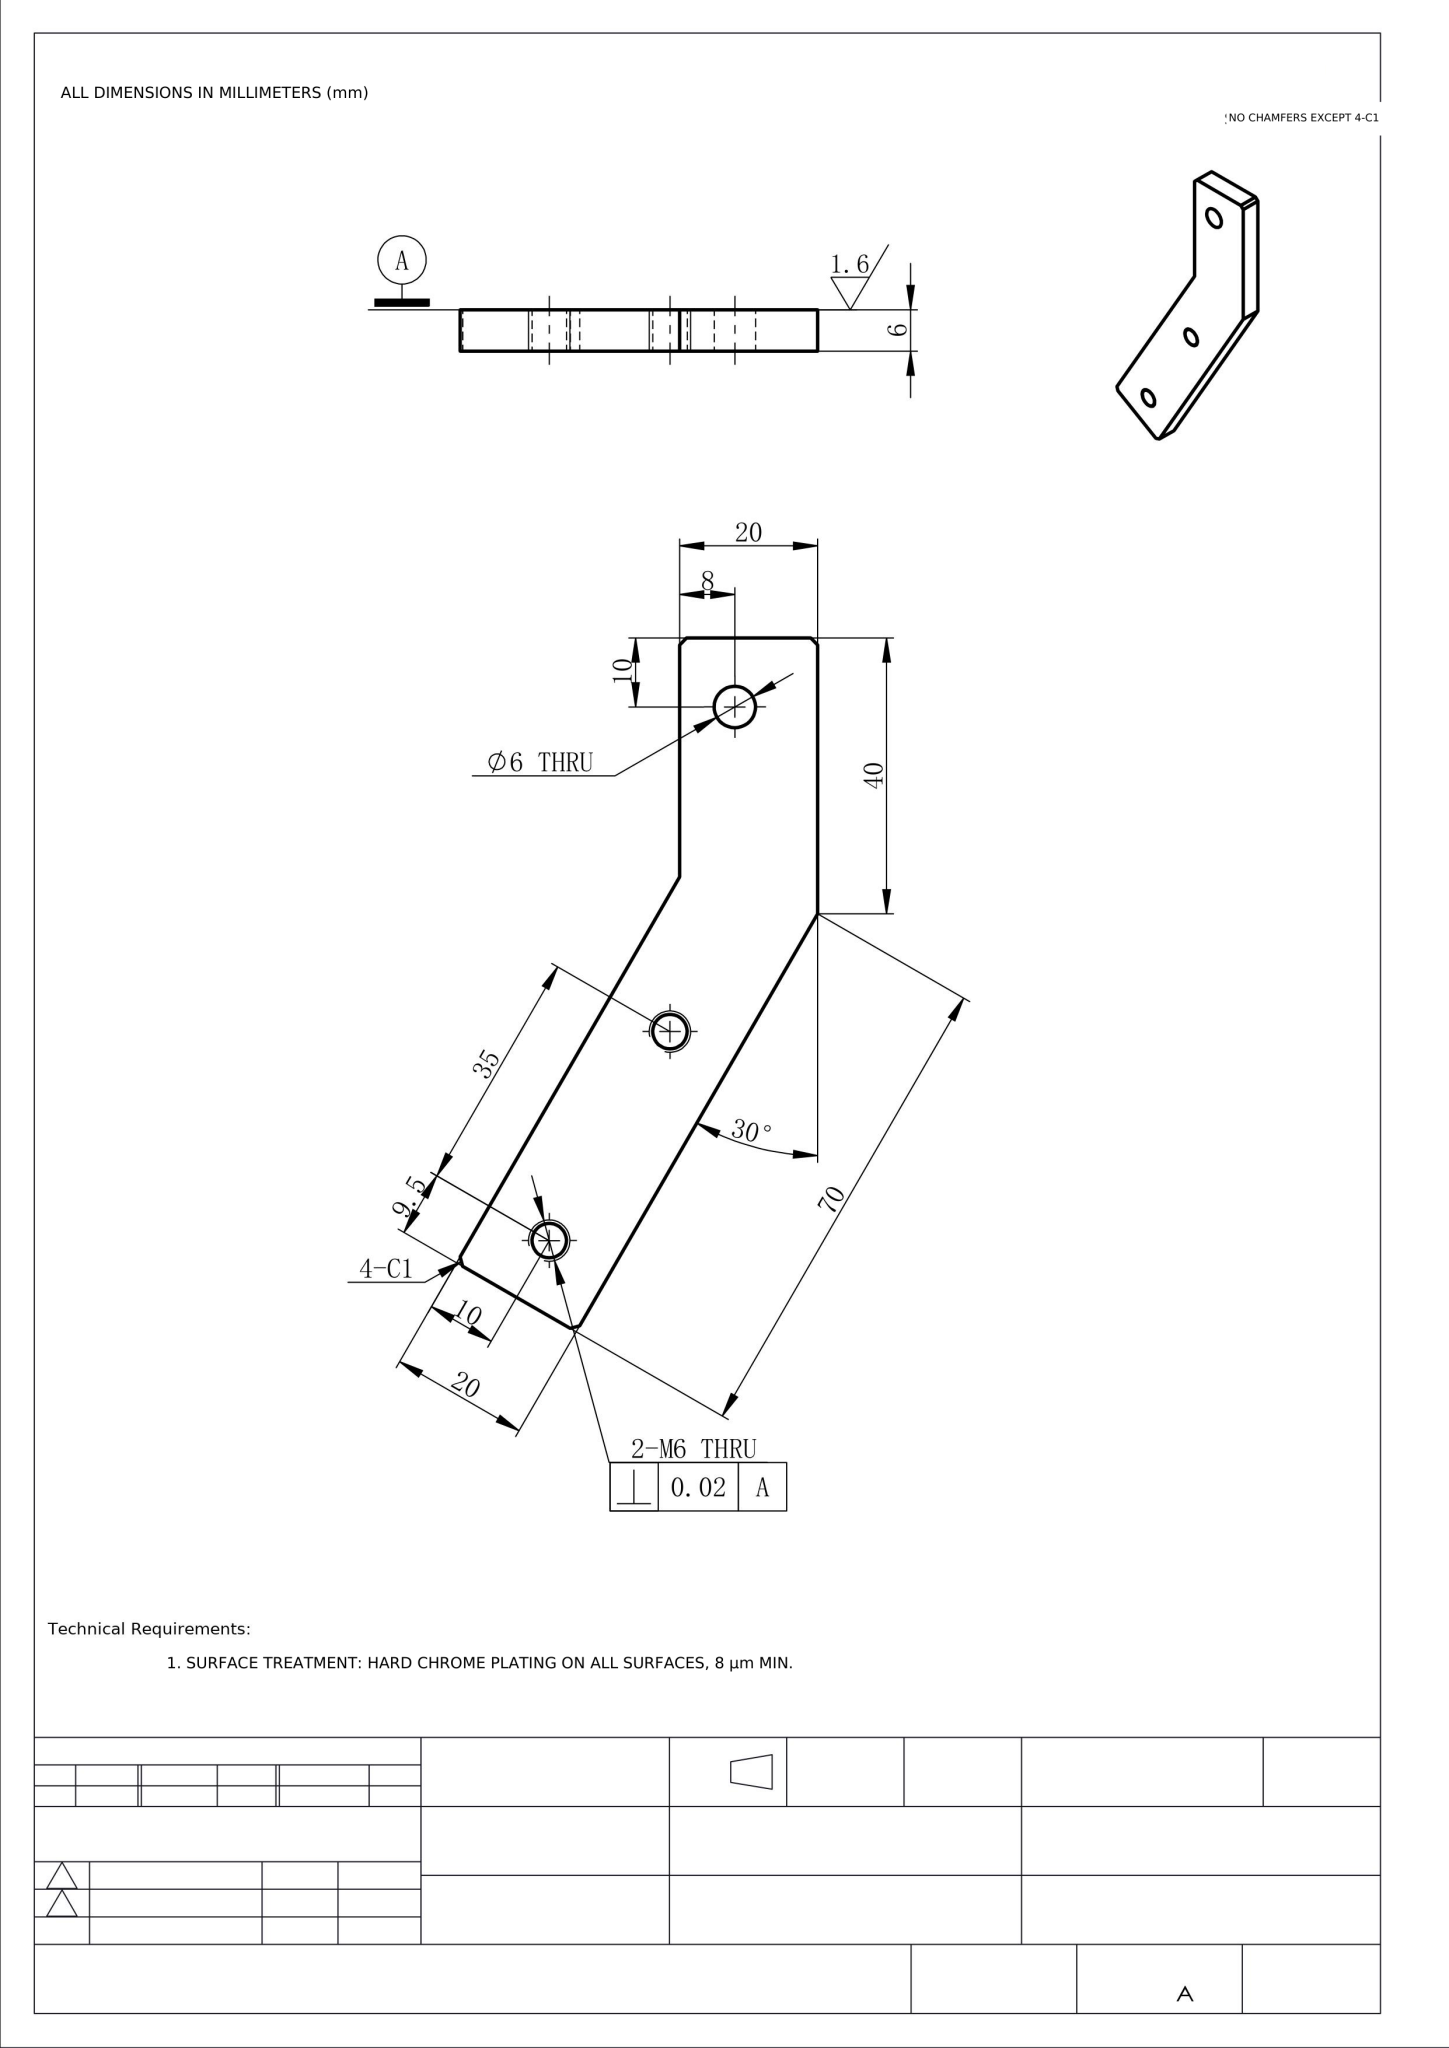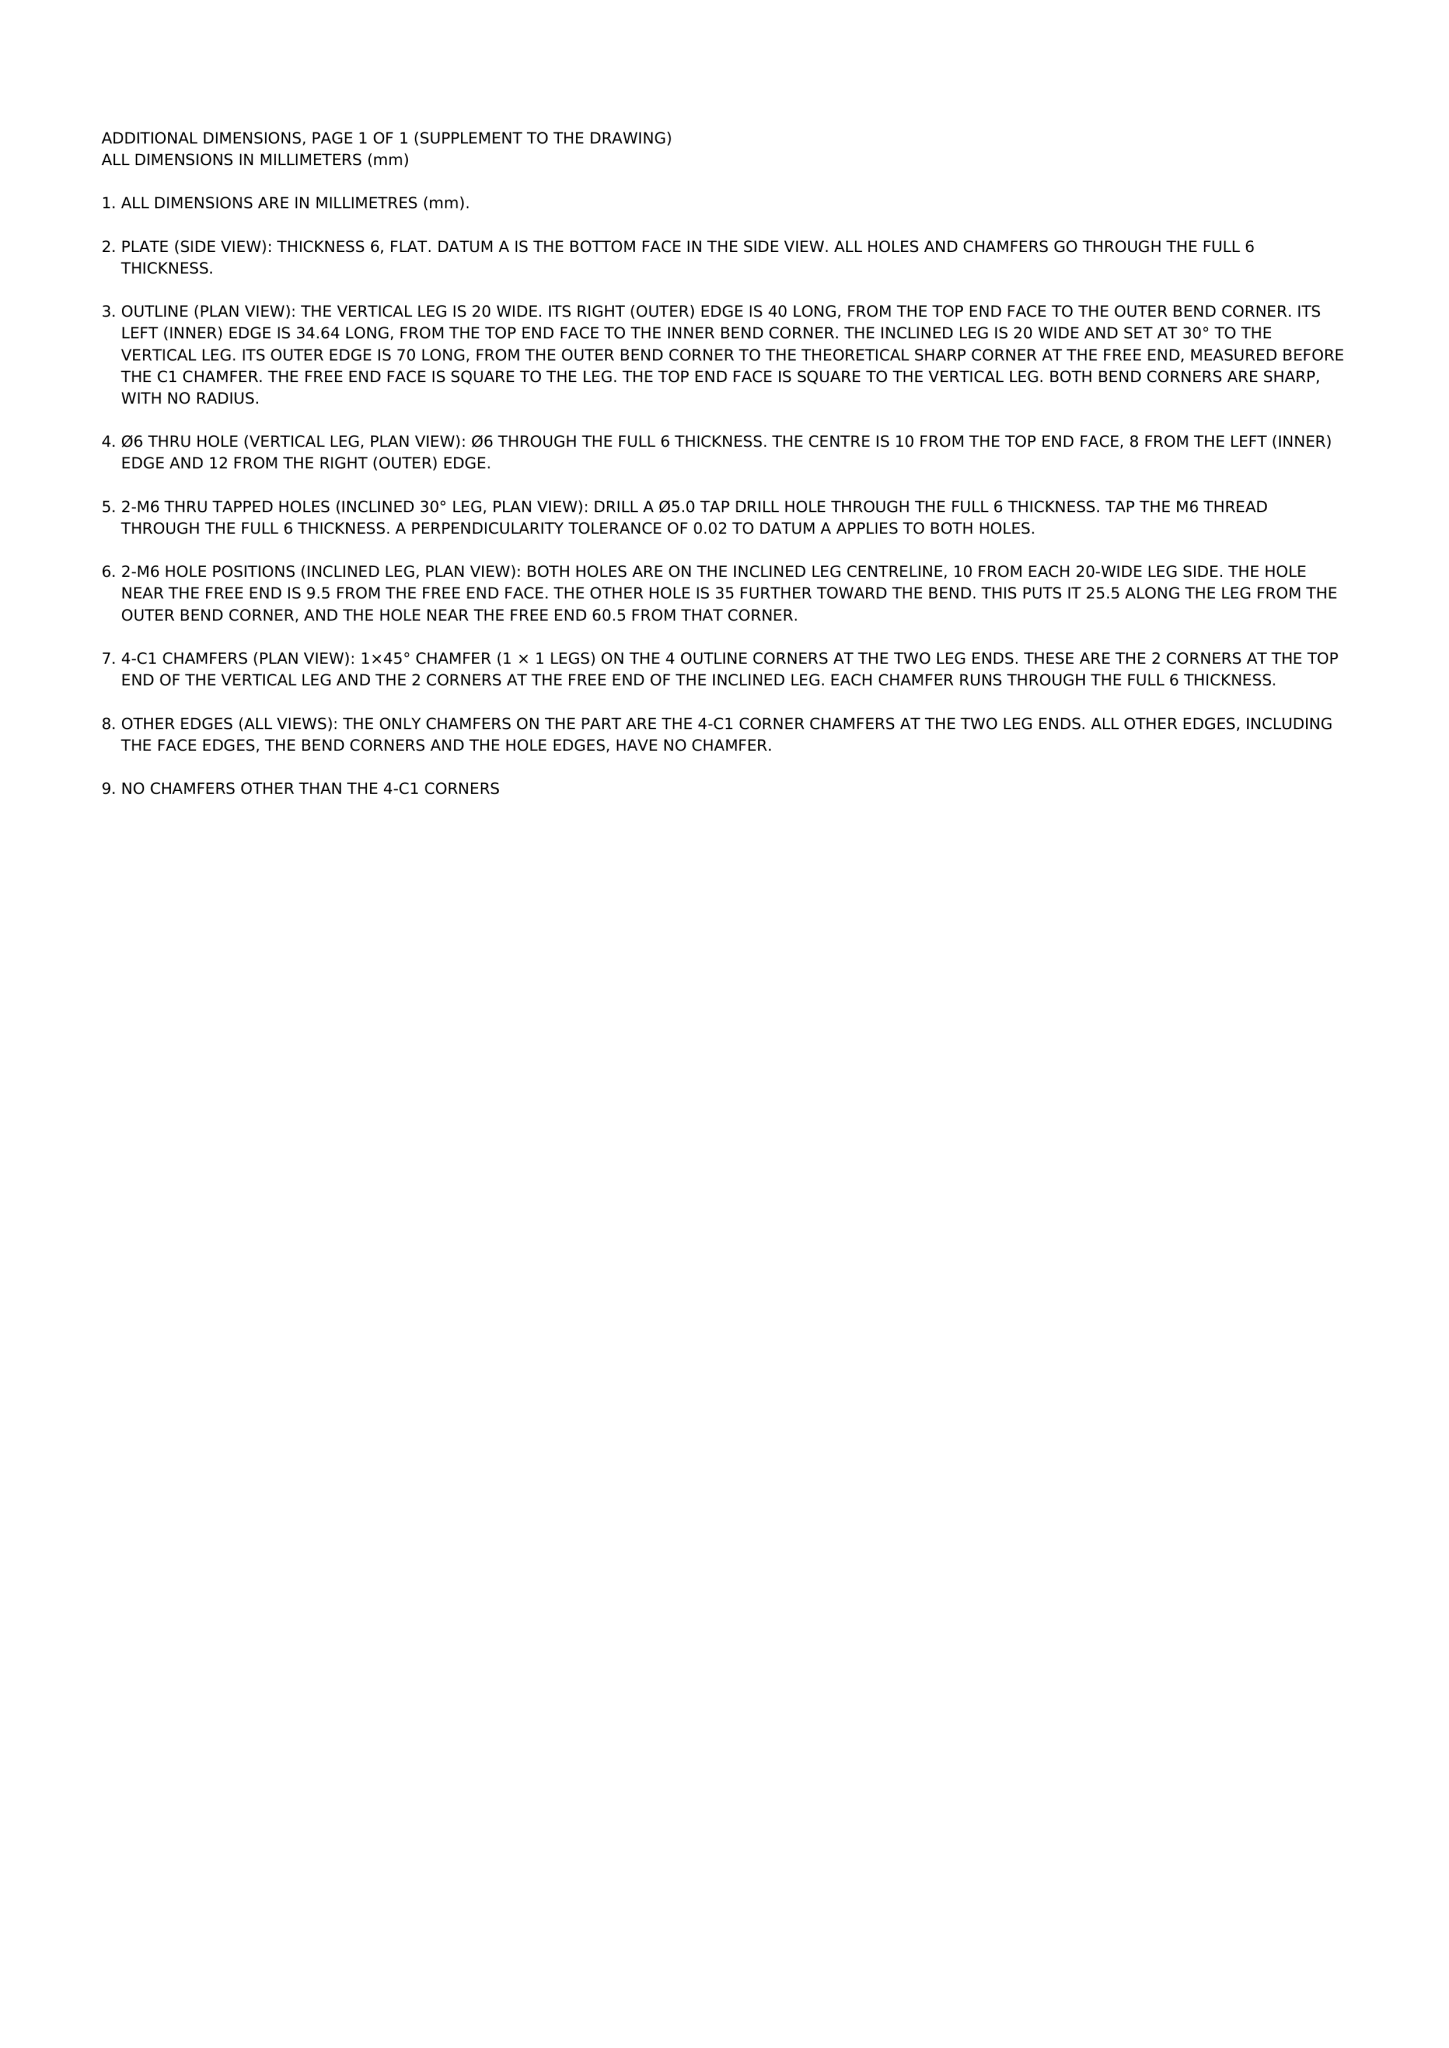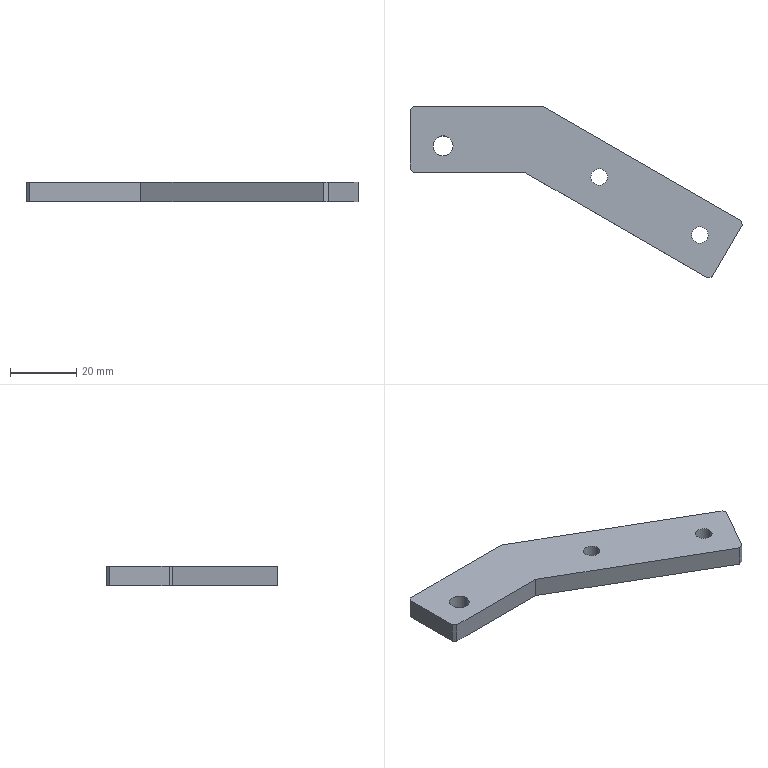Part | NX | mm | 1 solid | 18 faces | box 100.12 x 51.82 x 6 mm | volume 12140 mm3 | plane 12 | cylinder 6 | commonest cylinder face diameters 5 x4 6 x2
STEP:
#1=COLOUR_RGB('',0.7961,0.8235,0.9373);
#2=FILL_AREA_STYLE_COLOUR('',#1);
#3=FILL_AREA_STYLE('',(#2));
#4=SURFACE_STYLE_FILL_AREA(#3);
#5=SURFACE_SIDE_STYLE('',(#4));
#6=SURFACE_STYLE_USAGE(.BOTH.,#5);
#7=PRESENTATION_STYLE_ASSIGNMENT((#6));
#8=CARTESIAN_POINT('',(54.584,-21.41,-3.));
#9=VERTEX_POINT('',#8);
#10=CARTESIAN_POINT('',(59.584,-21.41,-3.));
#11=VERTEX_POINT('',#10);
#12=CARTESIAN_POINT('',(57.084,-21.41,-3.));
#13=DIRECTION('',(0.,0.,1.));
#14=DIRECTION('',(1.,0.,0.));
#15=AXIS2_PLACEMENT_3D('',#12,#13,#14);
#16=CIRCLE('',#15,2.5);
#17=EDGE_CURVE('',#9,#11,#16,.T.);
#18=ORIENTED_EDGE('',*,*,#17,.F.);
#19=CARTESIAN_POINT('',(54.584,-21.41,3.));
#20=VERTEX_POINT('',#19);
#21=CARTESIAN_POINT('',(54.584,-21.41,3.));
#22=DIRECTION('',(0.,0.,1.));
#23=VECTOR('',#22,1000.);
#24=LINE('',#21,#23);
#25=EDGE_CURVE('',#9,#20,#24,.T.);
#26=ORIENTED_EDGE('',*,*,#25,.T.);
#27=CARTESIAN_POINT('',(59.584,-21.41,3.));
#28=VERTEX_POINT('',#27);
#29=CARTESIAN_POINT('',(57.084,-21.41,3.));
#30=DIRECTION('',(0.,0.,1.));
#31=DIRECTION('',(1.,0.,0.));
#32=AXIS2_PLACEMENT_3D('',#29,#30,#31);
#33=CIRCLE('',#32,2.5);
#34=EDGE_CURVE('',#20,#28,#33,.T.);
#35=ORIENTED_EDGE('',*,*,#34,.T.);
#36=CARTESIAN_POINT('',(59.584,-21.41,3.));
#37=DIRECTION('',(0.,0.,1.));
#38=VECTOR('',#37,1000.);
#39=LINE('',#36,#38);
#40=EDGE_CURVE('',#11,#28,#39,.T.);
#41=ORIENTED_EDGE('',*,*,#40,.F.);
#42=EDGE_LOOP('',(#18,#26,#35,#41));
#43=FACE_OUTER_BOUND('',#42,.T.);
#44=CARTESIAN_POINT('',(57.084,-21.41,3.));
#45=DIRECTION('',(0.,0.,1.));
#46=DIRECTION('',(1.,0.,0.));
#47=AXIS2_PLACEMENT_3D('',#44,#45,#46);
#48=CYLINDRICAL_SURFACE('',#47,2.5);
#49=ADVANCED_FACE('',(#43),#48,.F.);
#50=CARTESIAN_POINT('',(84.895,-38.91,-3.));
#51=VERTEX_POINT('',#50);
#52=CARTESIAN_POINT('',(89.895,-38.91,-3.));
#53=VERTEX_POINT('',#52);
#54=CARTESIAN_POINT('',(87.395,-38.91,-3.));
#55=DIRECTION('',(0.,0.,1.));
#56=DIRECTION('',(1.,0.,0.));
#57=AXIS2_PLACEMENT_3D('',#54,#55,#56);
#58=CIRCLE('',#57,2.5);
#59=EDGE_CURVE('',#51,#53,#58,.T.);
#60=ORIENTED_EDGE('',*,*,#59,.F.);
#61=CARTESIAN_POINT('',(84.895,-38.91,3.));
#62=VERTEX_POINT('',#61);
#63=CARTESIAN_POINT('',(84.895,-38.91,3.));
#64=DIRECTION('',(0.,0.,1.));
#65=VECTOR('',#64,1000.);
#66=LINE('',#63,#65);
#67=EDGE_CURVE('',#51,#62,#66,.T.);
#68=ORIENTED_EDGE('',*,*,#67,.T.);
#69=CARTESIAN_POINT('',(89.895,-38.91,3.));
#70=VERTEX_POINT('',#69);
#71=CARTESIAN_POINT('',(87.395,-38.91,3.));
#72=DIRECTION('',(0.,0.,1.));
#73=DIRECTION('',(1.,0.,0.));
#74=AXIS2_PLACEMENT_3D('',#71,#72,#73);
#75=CIRCLE('',#74,2.5);
#76=EDGE_CURVE('',#62,#70,#75,.T.);
#77=ORIENTED_EDGE('',*,*,#76,.T.);
#78=CARTESIAN_POINT('',(89.895,-38.91,3.));
#79=DIRECTION('',(0.,0.,1.));
#80=VECTOR('',#79,1000.);
#81=LINE('',#78,#80);
#82=EDGE_CURVE('',#53,#70,#81,.T.);
#83=ORIENTED_EDGE('',*,*,#82,.F.);
#84=EDGE_LOOP('',(#60,#68,#77,#83));
#85=FACE_OUTER_BOUND('',#84,.T.);
#86=CARTESIAN_POINT('',(87.395,-38.91,3.));
#87=DIRECTION('',(0.,0.,1.));
#88=DIRECTION('',(1.,0.,0.));
#89=AXIS2_PLACEMENT_3D('',#86,#87,#88);
#90=CYLINDRICAL_SURFACE('',#89,2.5);
#91=ADVANCED_FACE('',(#85),#90,.F.);
#92=CARTESIAN_POINT('',(7.,-12.,-3.));
#93=VERTEX_POINT('',#92);
#94=CARTESIAN_POINT('',(13.,-12.,-3.));
#95=VERTEX_POINT('',#94);
#96=CARTESIAN_POINT('',(10.,-12.,-3.));
#97=DIRECTION('',(0.,0.,1.));
#98=DIRECTION('',(1.,0.,0.));
#99=AXIS2_PLACEMENT_3D('',#96,#97,#98);
#100=CIRCLE('',#99,3.);
#101=EDGE_CURVE('',#93,#95,#100,.T.);
#102=ORIENTED_EDGE('',*,*,#101,.F.);
#103=CARTESIAN_POINT('',(7.,-12.,3.));
#104=VERTEX_POINT('',#103);
#105=CARTESIAN_POINT('',(7.,-12.,-3.));
#106=DIRECTION('',(0.,0.,1.));
#107=VECTOR('',#106,1000.);
#108=LINE('',#105,#107);
#109=EDGE_CURVE('',#93,#104,#108,.T.);
#110=ORIENTED_EDGE('',*,*,#109,.T.);
#111=CARTESIAN_POINT('',(13.,-12.,3.));
#112=VERTEX_POINT('',#111);
#113=CARTESIAN_POINT('',(10.,-12.,3.));
#114=DIRECTION('',(0.,0.,1.));
#115=DIRECTION('',(1.,0.,0.));
#116=AXIS2_PLACEMENT_3D('',#113,#114,#115);
#117=CIRCLE('',#116,3.);
#118=EDGE_CURVE('',#104,#112,#117,.T.);
#119=ORIENTED_EDGE('',*,*,#118,.T.);
#120=CARTESIAN_POINT('',(13.,-12.,-3.));
#121=DIRECTION('',(0.,0.,1.));
#122=VECTOR('',#121,1000.);
#123=LINE('',#120,#122);
#124=EDGE_CURVE('',#95,#112,#123,.T.);
#125=ORIENTED_EDGE('',*,*,#124,.F.);
#126=EDGE_LOOP('',(#102,#110,#119,#125));
#127=FACE_OUTER_BOUND('',#126,.T.);
#128=CARTESIAN_POINT('',(10.,-12.,-3.));
#129=DIRECTION('',(0.,0.,1.));
#130=DIRECTION('',(1.,0.,0.));
#131=AXIS2_PLACEMENT_3D('',#128,#129,#130);
#132=CYLINDRICAL_SURFACE('',#131,3.);
#133=ADVANCED_FACE('',(#127),#132,.F.);
#134=CARTESIAN_POINT('',(0.,-1.,-3.));
#135=VERTEX_POINT('',#134);
#136=CARTESIAN_POINT('',(0.,-19.,-3.));
#137=VERTEX_POINT('',#136);
#138=CARTESIAN_POINT('',(0.,0.,-3.));
#139=DIRECTION('',(0.,-1.,0.));
#140=VECTOR('',#139,1000.);
#141=LINE('',#138,#140);
#142=EDGE_CURVE('',#135,#137,#141,.T.);
#143=ORIENTED_EDGE('',*,*,#142,.T.);
#144=CARTESIAN_POINT('',(0.,-19.,3.));
#145=VERTEX_POINT('',#144);
#146=CARTESIAN_POINT('',(0.,-19.,3.));
#147=DIRECTION('',(0.,0.,1.));
#148=VECTOR('',#147,1000.);
#149=LINE('',#146,#148);
#150=EDGE_CURVE('',#137,#145,#149,.T.);
#151=ORIENTED_EDGE('',*,*,#150,.T.);
#152=CARTESIAN_POINT('',(0.,-1.,3.));
#153=VERTEX_POINT('',#152);
#154=CARTESIAN_POINT('',(0.,0.,3.));
#155=DIRECTION('',(0.,-1.,0.));
#156=VECTOR('',#155,1000.);
#157=LINE('',#154,#156);
#158=EDGE_CURVE('',#153,#145,#157,.T.);
#159=ORIENTED_EDGE('',*,*,#158,.F.);
#160=CARTESIAN_POINT('',(0.,-1.,3.));
#161=DIRECTION('',(0.,0.,-1.));
#162=VECTOR('',#161,1000.);
#163=LINE('',#160,#162);
#164=EDGE_CURVE('',#153,#135,#163,.T.);
#165=ORIENTED_EDGE('',*,*,#164,.T.);
#166=EDGE_LOOP('',(#143,#151,#159,#165));
#167=FACE_OUTER_BOUND('',#166,.T.);
#168=CARTESIAN_POINT('',(0.,0.,3.));
#169=DIRECTION('',(1.,0.,0.));
#170=DIRECTION('',(-0.,1.,0.));
#171=AXIS2_PLACEMENT_3D('',#168,#169,#170);
#172=PLANE('',#171);
#173=ADVANCED_FACE('',(#167),#172,.F.);
#174=CARTESIAN_POINT('',(1.,-20.,3.));
#175=VERTEX_POINT('',#174);
#176=CARTESIAN_POINT('',(34.641,-20.,3.));
#177=VERTEX_POINT('',#176);
#178=CARTESIAN_POINT('',(0.,-20.,3.));
#179=DIRECTION('',(1.,0.,0.));
#180=VECTOR('',#179,1000.);
#181=LINE('',#178,#180);
#182=EDGE_CURVE('',#175,#177,#181,.T.);
#183=ORIENTED_EDGE('',*,*,#182,.F.);
#184=CARTESIAN_POINT('',(1.,-20.,-3.));
#185=VERTEX_POINT('',#184);
#186=CARTESIAN_POINT('',(1.,-20.,3.));
#187=DIRECTION('',(0.,0.,-1.));
#188=VECTOR('',#187,1000.);
#189=LINE('',#186,#188);
#190=EDGE_CURVE('',#175,#185,#189,.T.);
#191=ORIENTED_EDGE('',*,*,#190,.T.);
#192=CARTESIAN_POINT('',(34.641,-20.,-3.));
#193=VERTEX_POINT('',#192);
#194=CARTESIAN_POINT('',(0.,-20.,-3.));
#195=DIRECTION('',(1.,0.,0.));
#196=VECTOR('',#195,1000.);
#197=LINE('',#194,#196);
#198=EDGE_CURVE('',#185,#193,#197,.T.);
#199=ORIENTED_EDGE('',*,*,#198,.T.);
#200=CARTESIAN_POINT('',(34.641,-20.,3.));
#201=DIRECTION('',(0.,0.,-1.));
#202=VECTOR('',#201,1000.);
#203=LINE('',#200,#202);
#204=EDGE_CURVE('',#177,#193,#203,.T.);
#205=ORIENTED_EDGE('',*,*,#204,.F.);
#206=EDGE_LOOP('',(#183,#191,#199,#205));
#207=FACE_OUTER_BOUND('',#206,.T.);
#208=CARTESIAN_POINT('',(0.,-20.,3.));
#209=DIRECTION('',(0.,1.,0.));
#210=DIRECTION('',(0.,0.,1.));
#211=AXIS2_PLACEMENT_3D('',#208,#209,#210);
#212=PLANE('',#211);
#213=ADVANCED_FACE('',(#207),#212,.F.);
#214=CARTESIAN_POINT('',(89.756,-51.821,-3.));
#215=VERTEX_POINT('',#214);
#216=CARTESIAN_POINT('',(34.641,-20.,-3.));
#217=DIRECTION('',(0.866,-0.5,0.));
#218=VECTOR('',#217,1000.);
#219=LINE('',#216,#218);
#220=EDGE_CURVE('',#193,#215,#219,.T.);
#221=ORIENTED_EDGE('',*,*,#220,.T.);
#222=CARTESIAN_POINT('',(89.756,-51.821,3.));
#223=VERTEX_POINT('',#222);
#224=CARTESIAN_POINT('',(89.756,-51.821,3.));
#225=DIRECTION('',(0.,0.,1.));
#226=VECTOR('',#225,1000.);
#227=LINE('',#224,#226);
#228=EDGE_CURVE('',#215,#223,#227,.T.);
#229=ORIENTED_EDGE('',*,*,#228,.T.);
#230=CARTESIAN_POINT('',(34.641,-20.,3.));
#231=DIRECTION('',(0.866,-0.5,0.));
#232=VECTOR('',#231,1000.);
#233=LINE('',#230,#232);
#234=EDGE_CURVE('',#177,#223,#233,.T.);
#235=ORIENTED_EDGE('',*,*,#234,.F.);
#236=ORIENTED_EDGE('',*,*,#204,.T.);
#237=EDGE_LOOP('',(#221,#229,#235,#236));
#238=FACE_OUTER_BOUND('',#237,.T.);
#239=CARTESIAN_POINT('',(34.641,-20.,3.));
#240=DIRECTION('',(0.5,0.866,0.));
#241=DIRECTION('',(-0.866,0.5,0.));
#242=AXIS2_PLACEMENT_3D('',#239,#240,#241);
#243=PLANE('',#242);
#244=ADVANCED_FACE('',(#238),#243,.F.);
#245=CARTESIAN_POINT('',(91.122,-51.454,3.));
#246=VERTEX_POINT('',#245);
#247=CARTESIAN_POINT('',(100.122,-35.866,3.));
#248=VERTEX_POINT('',#247);
#249=CARTESIAN_POINT('',(90.622,-52.321,3.));
#250=DIRECTION('',(0.5,0.866,0.));
#251=VECTOR('',#250,1000.);
#252=LINE('',#249,#251);
#253=EDGE_CURVE('',#246,#248,#252,.T.);
#254=ORIENTED_EDGE('',*,*,#253,.F.);
#255=CARTESIAN_POINT('',(91.122,-51.454,-3.));
#256=VERTEX_POINT('',#255);
#257=CARTESIAN_POINT('',(91.122,-51.454,3.));
#258=DIRECTION('',(0.,0.,-1.));
#259=VECTOR('',#258,1000.);
#260=LINE('',#257,#259);
#261=EDGE_CURVE('',#246,#256,#260,.T.);
#262=ORIENTED_EDGE('',*,*,#261,.T.);
#263=CARTESIAN_POINT('',(100.122,-35.866,-3.));
#264=VERTEX_POINT('',#263);
#265=CARTESIAN_POINT('',(90.622,-52.321,-3.));
#266=DIRECTION('',(0.5,0.866,0.));
#267=VECTOR('',#266,1000.);
#268=LINE('',#265,#267);
#269=EDGE_CURVE('',#256,#264,#268,.T.);
#270=ORIENTED_EDGE('',*,*,#269,.T.);
#271=CARTESIAN_POINT('',(100.122,-35.866,3.));
#272=DIRECTION('',(0.,0.,1.));
#273=VECTOR('',#272,1000.);
#274=LINE('',#271,#273);
#275=EDGE_CURVE('',#264,#248,#274,.T.);
#276=ORIENTED_EDGE('',*,*,#275,.T.);
#277=EDGE_LOOP('',(#254,#262,#270,#276));
#278=FACE_OUTER_BOUND('',#277,.T.);
#279=CARTESIAN_POINT('',(90.622,-52.321,3.));
#280=DIRECTION('',(-0.866,0.5,0.));
#281=DIRECTION('',(-0.5,-0.866,0.));
#282=AXIS2_PLACEMENT_3D('',#279,#280,#281);
#283=PLANE('',#282);
#284=ADVANCED_FACE('',(#278),#283,.F.);
#285=CARTESIAN_POINT('',(99.756,-34.5,3.));
#286=VERTEX_POINT('',#285);
#287=CARTESIAN_POINT('',(40.,0.,3.));
#288=VERTEX_POINT('',#287);
#289=CARTESIAN_POINT('',(40.,0.,3.));
#290=DIRECTION('',(-0.866,0.5,0.));
#291=VECTOR('',#290,1000.);
#292=LINE('',#289,#291);
#293=EDGE_CURVE('',#286,#288,#292,.T.);
#294=ORIENTED_EDGE('',*,*,#293,.F.);
#295=CARTESIAN_POINT('',(99.756,-34.5,-3.));
#296=VERTEX_POINT('',#295);
#297=CARTESIAN_POINT('',(99.756,-34.5,3.));
#298=DIRECTION('',(0.,0.,-1.));
#299=VECTOR('',#298,1000.);
#300=LINE('',#297,#299);
#301=EDGE_CURVE('',#286,#296,#300,.T.);
#302=ORIENTED_EDGE('',*,*,#301,.T.);
#303=CARTESIAN_POINT('',(40.,0.,-3.));
#304=VERTEX_POINT('',#303);
#305=CARTESIAN_POINT('',(40.,0.,-3.));
#306=DIRECTION('',(-0.866,0.5,0.));
#307=VECTOR('',#306,1000.);
#308=LINE('',#305,#307);
#309=EDGE_CURVE('',#296,#304,#308,.T.);
#310=ORIENTED_EDGE('',*,*,#309,.T.);
#311=CARTESIAN_POINT('',(40.,0.,3.));
#312=DIRECTION('',(0.,0.,-1.));
#313=VECTOR('',#312,1000.);
#314=LINE('',#311,#313);
#315=EDGE_CURVE('',#288,#304,#314,.T.);
#316=ORIENTED_EDGE('',*,*,#315,.F.);
#317=EDGE_LOOP('',(#294,#302,#310,#316));
#318=FACE_OUTER_BOUND('',#317,.T.);
#319=CARTESIAN_POINT('',(40.,0.,3.));
#320=DIRECTION('',(-0.5,-0.866,0.));
#321=DIRECTION('',(0.866,-0.5,0.));
#322=AXIS2_PLACEMENT_3D('',#319,#320,#321);
#323=PLANE('',#322);
#324=ADVANCED_FACE('',(#318),#323,.F.);
#325=CARTESIAN_POINT('',(1.,0.,-3.));
#326=VERTEX_POINT('',#325);
#327=CARTESIAN_POINT('',(0.,0.,-3.));
#328=DIRECTION('',(-1.,0.,0.));
#329=VECTOR('',#328,1000.);
#330=LINE('',#327,#329);
#331=EDGE_CURVE('',#304,#326,#330,.T.);
#332=ORIENTED_EDGE('',*,*,#331,.T.);
#333=CARTESIAN_POINT('',(1.,0.,3.));
#334=VERTEX_POINT('',#333);
#335=CARTESIAN_POINT('',(1.,0.,3.));
#336=DIRECTION('',(0.,0.,1.));
#337=VECTOR('',#336,1000.);
#338=LINE('',#335,#337);
#339=EDGE_CURVE('',#326,#334,#338,.T.);
#340=ORIENTED_EDGE('',*,*,#339,.T.);
#341=CARTESIAN_POINT('',(0.,0.,3.));
#342=DIRECTION('',(-1.,0.,0.));
#343=VECTOR('',#342,1000.);
#344=LINE('',#341,#343);
#345=EDGE_CURVE('',#288,#334,#344,.T.);
#346=ORIENTED_EDGE('',*,*,#345,.F.);
#347=ORIENTED_EDGE('',*,*,#315,.T.);
#348=EDGE_LOOP('',(#332,#340,#346,#347));
#349=FACE_OUTER_BOUND('',#348,.T.);
#350=CARTESIAN_POINT('',(0.,0.,3.));
#351=DIRECTION('',(0.,-1.,0.));
#352=DIRECTION('',(0.,0.,-1.));
#353=AXIS2_PLACEMENT_3D('',#350,#351,#352);
#354=PLANE('',#353);
#355=ADVANCED_FACE('',(#349),#354,.F.);
#356=CARTESIAN_POINT('',(57.084,-21.41,3.));
#357=DIRECTION('',(0.,0.,1.));
#358=DIRECTION('',(1.,0.,0.));
#359=AXIS2_PLACEMENT_3D('',#356,#357,#358);
#360=CIRCLE('',#359,2.5);
#361=EDGE_CURVE('',#28,#20,#360,.T.);
#362=ORIENTED_EDGE('',*,*,#361,.F.);
#363=ORIENTED_EDGE('',*,*,#34,.F.);
#364=EDGE_LOOP('',(#362,#363));
#365=FACE_BOUND('',#364,.T.);
#366=CARTESIAN_POINT('',(87.395,-38.91,3.));
#367=DIRECTION('',(0.,0.,1.));
#368=DIRECTION('',(1.,0.,0.));
#369=AXIS2_PLACEMENT_3D('',#366,#367,#368);
#370=CIRCLE('',#369,2.5);
#371=EDGE_CURVE('',#70,#62,#370,.T.);
#372=ORIENTED_EDGE('',*,*,#371,.F.);
#373=ORIENTED_EDGE('',*,*,#76,.F.);
#374=EDGE_LOOP('',(#372,#373));
#375=FACE_BOUND('',#374,.T.);
#376=CARTESIAN_POINT('',(10.,-12.,3.));
#377=DIRECTION('',(0.,0.,1.));
#378=DIRECTION('',(1.,0.,0.));
#379=AXIS2_PLACEMENT_3D('',#376,#377,#378);
#380=CIRCLE('',#379,3.);
#381=EDGE_CURVE('',#112,#104,#380,.T.);
#382=ORIENTED_EDGE('',*,*,#381,.F.);
#383=ORIENTED_EDGE('',*,*,#118,.F.);
#384=EDGE_LOOP('',(#382,#383));
#385=FACE_BOUND('',#384,.T.);
#386=ORIENTED_EDGE('',*,*,#234,.T.);
#387=CARTESIAN_POINT('',(13.968,-72.128,3.));
#388=DIRECTION('',(0.9659,0.2588,0.));
#389=VECTOR('',#388,1000.);
#390=LINE('',#387,#389);
#391=EDGE_CURVE('',#223,#246,#390,.T.);
#392=ORIENTED_EDGE('',*,*,#391,.T.);
#393=ORIENTED_EDGE('',*,*,#253,.T.);
#394=CARTESIAN_POINT('',(89.448,3.968,3.));
#395=DIRECTION('',(-0.2588,0.9659,0.));
#396=VECTOR('',#395,1000.);
#397=LINE('',#394,#396);
#398=EDGE_CURVE('',#248,#286,#397,.T.);
#399=ORIENTED_EDGE('',*,*,#398,.T.);
#400=ORIENTED_EDGE('',*,*,#293,.T.);
#401=ORIENTED_EDGE('',*,*,#345,.T.);
#402=CARTESIAN_POINT('',(-9.5,-10.5,3.));
#403=DIRECTION('',(-0.7071,-0.7071,0.));
#404=VECTOR('',#403,1000.);
#405=LINE('',#402,#404);
#406=EDGE_CURVE('',#334,#153,#405,.T.);
#407=ORIENTED_EDGE('',*,*,#406,.T.);
#408=ORIENTED_EDGE('',*,*,#158,.T.);
#409=CARTESIAN_POINT('',(0.5,-19.5,3.));
#410=DIRECTION('',(0.7071,-0.7071,0.));
#411=VECTOR('',#410,1000.);
#412=LINE('',#409,#411);
#413=EDGE_CURVE('',#145,#175,#412,.T.);
#414=ORIENTED_EDGE('',*,*,#413,.T.);
#415=ORIENTED_EDGE('',*,*,#182,.T.);
#416=EDGE_LOOP('',(#386,#392,#393,#399,#400,#401,#407,#408,#414,#415));
#417=FACE_OUTER_BOUND('',#416,.T.);
#418=CARTESIAN_POINT('',(0.,-20.,3.));
#419=DIRECTION('',(0.,0.,1.));
#420=DIRECTION('',(1.,0.,0.));
#421=AXIS2_PLACEMENT_3D('',#418,#419,#420);
#422=PLANE('',#421);
#423=ADVANCED_FACE('',(#365,#375,#385,#417),#422,.T.);
#424=CARTESIAN_POINT('',(57.084,-21.41,-3.));
#425=DIRECTION('',(0.,0.,1.));
#426=DIRECTION('',(1.,0.,0.));
#427=AXIS2_PLACEMENT_3D('',#424,#425,#426);
#428=CIRCLE('',#427,2.5);
#429=EDGE_CURVE('',#11,#9,#428,.T.);
#430=ORIENTED_EDGE('',*,*,#429,.T.);
#431=ORIENTED_EDGE('',*,*,#17,.T.);
#432=EDGE_LOOP('',(#430,#431));
#433=FACE_BOUND('',#432,.T.);
#434=CARTESIAN_POINT('',(87.395,-38.91,-3.));
#435=DIRECTION('',(0.,0.,1.));
#436=DIRECTION('',(1.,0.,0.));
#437=AXIS2_PLACEMENT_3D('',#434,#435,#436);
#438=CIRCLE('',#437,2.5);
#439=EDGE_CURVE('',#53,#51,#438,.T.);
#440=ORIENTED_EDGE('',*,*,#439,.T.);
#441=ORIENTED_EDGE('',*,*,#59,.T.);
#442=EDGE_LOOP('',(#440,#441));
#443=FACE_BOUND('',#442,.T.);
#444=CARTESIAN_POINT('',(10.,-12.,-3.));
#445=DIRECTION('',(0.,0.,1.));
#446=DIRECTION('',(1.,0.,0.));
#447=AXIS2_PLACEMENT_3D('',#444,#445,#446);
#448=CIRCLE('',#447,3.);
#449=EDGE_CURVE('',#95,#93,#448,.T.);
#450=ORIENTED_EDGE('',*,*,#449,.T.);
#451=ORIENTED_EDGE('',*,*,#101,.T.);
#452=EDGE_LOOP('',(#450,#451));
#453=FACE_BOUND('',#452,.T.);
#454=ORIENTED_EDGE('',*,*,#269,.F.);
#455=CARTESIAN_POINT('',(91.122,-51.454,-3.));
#456=DIRECTION('',(-0.9659,-0.2588,0.));
#457=VECTOR('',#456,1000.);
#458=LINE('',#455,#457);
#459=EDGE_CURVE('',#256,#215,#458,.T.);
#460=ORIENTED_EDGE('',*,*,#459,.T.);
#461=ORIENTED_EDGE('',*,*,#220,.F.);
#462=ORIENTED_EDGE('',*,*,#198,.F.);
#463=CARTESIAN_POINT('',(1.,-20.,-3.));
#464=DIRECTION('',(-0.7071,0.7071,0.));
#465=VECTOR('',#464,1000.);
#466=LINE('',#463,#465);
#467=EDGE_CURVE('',#185,#137,#466,.T.);
#468=ORIENTED_EDGE('',*,*,#467,.T.);
#469=ORIENTED_EDGE('',*,*,#142,.F.);
#470=CARTESIAN_POINT('',(0.,-1.,-3.));
#471=DIRECTION('',(0.7071,0.7071,0.));
#472=VECTOR('',#471,1000.);
#473=LINE('',#470,#472);
#474=EDGE_CURVE('',#135,#326,#473,.T.);
#475=ORIENTED_EDGE('',*,*,#474,.T.);
#476=ORIENTED_EDGE('',*,*,#331,.F.);
#477=ORIENTED_EDGE('',*,*,#309,.F.);
#478=CARTESIAN_POINT('',(99.756,-34.5,-3.));
#479=DIRECTION('',(0.2588,-0.9659,0.));
#480=VECTOR('',#479,1000.);
#481=LINE('',#478,#480);
#482=EDGE_CURVE('',#296,#264,#481,.T.);
#483=ORIENTED_EDGE('',*,*,#482,.T.);
#484=EDGE_LOOP('',(#454,#460,#461,#462,#468,#469,#475,#476,#477,#483));
#485=FACE_OUTER_BOUND('',#484,.T.);
#486=CARTESIAN_POINT('',(0.,-20.,-3.));
#487=DIRECTION('',(0.,0.,1.));
#488=DIRECTION('',(1.,0.,0.));
#489=AXIS2_PLACEMENT_3D('',#486,#487,#488);
#490=PLANE('',#489);
#491=ADVANCED_FACE('',(#433,#443,#453,#485),#490,.F.);
#492=ORIENTED_EDGE('',*,*,#109,.F.);
#493=ORIENTED_EDGE('',*,*,#449,.F.);
#494=ORIENTED_EDGE('',*,*,#124,.T.);
#495=ORIENTED_EDGE('',*,*,#381,.T.);
#496=EDGE_LOOP('',(#492,#493,#494,#495));
#497=FACE_OUTER_BOUND('',#496,.T.);
#498=CARTESIAN_POINT('',(10.,-12.,-3.));
#499=DIRECTION('',(0.,0.,1.));
#500=DIRECTION('',(1.,0.,0.));
#501=AXIS2_PLACEMENT_3D('',#498,#499,#500);
#502=CYLINDRICAL_SURFACE('',#501,3.);
#503=ADVANCED_FACE('',(#497),#502,.F.);
#504=ORIENTED_EDGE('',*,*,#67,.F.);
#505=ORIENTED_EDGE('',*,*,#439,.F.);
#506=ORIENTED_EDGE('',*,*,#82,.T.);
#507=ORIENTED_EDGE('',*,*,#371,.T.);
#508=EDGE_LOOP('',(#504,#505,#506,#507));
#509=FACE_OUTER_BOUND('',#508,.T.);
#510=CARTESIAN_POINT('',(87.395,-38.91,3.));
#511=DIRECTION('',(0.,0.,1.));
#512=DIRECTION('',(1.,0.,0.));
#513=AXIS2_PLACEMENT_3D('',#510,#511,#512);
#514=CYLINDRICAL_SURFACE('',#513,2.5);
#515=ADVANCED_FACE('',(#509),#514,.F.);
#516=ORIENTED_EDGE('',*,*,#25,.F.);
#517=ORIENTED_EDGE('',*,*,#429,.F.);
#518=ORIENTED_EDGE('',*,*,#40,.T.);
#519=ORIENTED_EDGE('',*,*,#361,.T.);
#520=EDGE_LOOP('',(#516,#517,#518,#519));
#521=FACE_OUTER_BOUND('',#520,.T.);
#522=CARTESIAN_POINT('',(57.084,-21.41,3.));
#523=DIRECTION('',(0.,0.,1.));
#524=DIRECTION('',(1.,0.,0.));
#525=AXIS2_PLACEMENT_3D('',#522,#523,#524);
#526=CYLINDRICAL_SURFACE('',#525,2.5);
#527=ADVANCED_FACE('',(#521),#526,.F.);
#528=ORIENTED_EDGE('',*,*,#391,.F.);
#529=ORIENTED_EDGE('',*,*,#228,.F.);
#530=ORIENTED_EDGE('',*,*,#459,.F.);
#531=ORIENTED_EDGE('',*,*,#261,.F.);
#532=EDGE_LOOP('',(#528,#529,#530,#531));
#533=FACE_OUTER_BOUND('',#532,.T.);
#534=CARTESIAN_POINT('',(91.122,-51.454,3.));
#535=DIRECTION('',(-0.2588,0.9659,0.));
#536=DIRECTION('',(-0.9659,-0.2588,0.));
#537=AXIS2_PLACEMENT_3D('',#534,#535,#536);
#538=PLANE('',#537);
#539=ADVANCED_FACE('',(#533),#538,.F.);
#540=ORIENTED_EDGE('',*,*,#398,.F.);
#541=ORIENTED_EDGE('',*,*,#275,.F.);
#542=ORIENTED_EDGE('',*,*,#482,.F.);
#543=ORIENTED_EDGE('',*,*,#301,.F.);
#544=EDGE_LOOP('',(#540,#541,#542,#543));
#545=FACE_OUTER_BOUND('',#544,.T.);
#546=CARTESIAN_POINT('',(99.756,-34.5,3.));
#547=DIRECTION('',(-0.9659,-0.2588,0.));
#548=DIRECTION('',(0.2588,-0.9659,0.));
#549=AXIS2_PLACEMENT_3D('',#546,#547,#548);
#550=PLANE('',#549);
#551=ADVANCED_FACE('',(#545),#550,.F.);
#552=ORIENTED_EDGE('',*,*,#413,.F.);
#553=ORIENTED_EDGE('',*,*,#150,.F.);
#554=ORIENTED_EDGE('',*,*,#467,.F.);
#555=ORIENTED_EDGE('',*,*,#190,.F.);
#556=EDGE_LOOP('',(#552,#553,#554,#555));
#557=FACE_OUTER_BOUND('',#556,.T.);
#558=CARTESIAN_POINT('',(1.,-20.,3.));
#559=DIRECTION('',(0.7071,0.7071,0.));
#560=DIRECTION('',(-0.7071,0.7071,0.));
#561=AXIS2_PLACEMENT_3D('',#558,#559,#560);
#562=PLANE('',#561);
#563=ADVANCED_FACE('',(#557),#562,.F.);
#564=ORIENTED_EDGE('',*,*,#406,.F.);
#565=ORIENTED_EDGE('',*,*,#339,.F.);
#566=ORIENTED_EDGE('',*,*,#474,.F.);
#567=ORIENTED_EDGE('',*,*,#164,.F.);
#568=EDGE_LOOP('',(#564,#565,#566,#567));
#569=FACE_OUTER_BOUND('',#568,.T.);
#570=CARTESIAN_POINT('',(0.,-1.,3.));
#571=DIRECTION('',(0.7071,-0.7071,0.));
#572=DIRECTION('',(0.7071,0.7071,0.));
#573=AXIS2_PLACEMENT_3D('',#570,#571,#572);
#574=PLANE('',#573);
#575=ADVANCED_FACE('',(#569),#574,.F.);
#576=CLOSED_SHELL('',(#49,#91,#133,#173,#213,#244,#284,#324,#355,#423,#491,#503,#515,#527,#539,#551,#563,#575));
#577=MANIFOLD_SOLID_BREP('',#576);
#578=STYLED_ITEM('',(#7),#577);
#579=(LENGTH_UNIT()NAMED_UNIT(*)SI_UNIT(.MILLI.,.METRE.));
#580=UNCERTAINTY_MEASURE_WITH_UNIT(LENGTH_MEASURE(0.00001),#579,'','');
#581=(NAMED_UNIT(*)PLANE_ANGLE_UNIT()SI_UNIT($,.RADIAN.));
#582=(NAMED_UNIT(*)SI_UNIT($,.STERADIAN.)SOLID_ANGLE_UNIT());
#583=(GEOMETRIC_REPRESENTATION_CONTEXT(3)GLOBAL_UNCERTAINTY_ASSIGNED_CONTEXT((#580))GLOBAL_UNIT_ASSIGNED_CONTEXT((#579,#581,#582))REPRESENTATION_CONTEXT('',''));
#584=MECHANICAL_DESIGN_GEOMETRIC_PRESENTATION_REPRESENTATION('',(#578),#583);
#585=COLOUR_RGB('',0.7961,0.8235,0.9373);
#586=FILL_AREA_STYLE_COLOUR('',#585);
#587=FILL_AREA_STYLE('',(#586));
#588=SURFACE_STYLE_FILL_AREA(#587);
#589=SURFACE_SIDE_STYLE('',(#588));
#590=SURFACE_STYLE_USAGE(.BOTH.,#589);
#591=PRESENTATION_STYLE_ASSIGNMENT((#590));
#592=STYLED_ITEM('',(#591),#91);
#593=PRESENTATION_LAYER_ASSIGNMENT('','',(#592));
#594=COLOUR_RGB('',0.7961,0.8235,0.9373);
#595=FILL_AREA_STYLE_COLOUR('',#594);
#596=FILL_AREA_STYLE('',(#595));
#597=SURFACE_STYLE_FILL_AREA(#596);
#598=SURFACE_SIDE_STYLE('',(#597));
#599=SURFACE_STYLE_USAGE(.BOTH.,#598);
#600=PRESENTATION_STYLE_ASSIGNMENT((#599));
#601=STYLED_ITEM('',(#600),#527);
#602=PRESENTATION_LAYER_ASSIGNMENT('','',(#601));
#603=COLOUR_RGB('',0.7961,0.8235,0.9373);
#604=FILL_AREA_STYLE_COLOUR('',#603);
#605=FILL_AREA_STYLE('',(#604));
#606=SURFACE_STYLE_FILL_AREA(#605);
#607=SURFACE_SIDE_STYLE('',(#606));
#608=SURFACE_STYLE_USAGE(.BOTH.,#607);
#609=PRESENTATION_STYLE_ASSIGNMENT((#608));
#610=CARTESIAN_POINT('',(0.,0.,0.));
#611=DIRECTION('',(0.,0.,1.));
#612=DIRECTION('',(1.,0.,0.));
#613=AXIS2_PLACEMENT_3D('',#610,#611,#612);
#614=(LENGTH_UNIT()NAMED_UNIT(*)SI_UNIT(.MILLI.,.METRE.));
#615=UNCERTAINTY_MEASURE_WITH_UNIT(LENGTH_MEASURE(0.00001),#614,'','');
#616=(NAMED_UNIT(*)PLANE_ANGLE_UNIT()SI_UNIT($,.RADIAN.));
#617=(NAMED_UNIT(*)SI_UNIT($,.STERADIAN.)SOLID_ANGLE_UNIT());
#618=(GEOMETRIC_REPRESENTATION_CONTEXT(3)GLOBAL_UNCERTAINTY_ASSIGNED_CONTEXT((#615))GLOBAL_UNIT_ASSIGNED_CONTEXT((#614,#616,#617))REPRESENTATION_CONTEXT('',''));
#619=ADVANCED_BREP_SHAPE_REPRESENTATION('',(#577,#613),#618);
#620=STYLED_ITEM('',(#609),#619);
#621=PRESENTATION_LAYER_ASSIGNMENT('','',(#620));
#622=(LENGTH_UNIT()NAMED_UNIT(*)SI_UNIT(.MILLI.,.METRE.));
#623=UNCERTAINTY_MEASURE_WITH_UNIT(LENGTH_MEASURE(0.00001),#622,'','');
#624=(NAMED_UNIT(*)PLANE_ANGLE_UNIT()SI_UNIT($,.RADIAN.));
#625=(NAMED_UNIT(*)SI_UNIT($,.STERADIAN.)SOLID_ANGLE_UNIT());
#626=(GEOMETRIC_REPRESENTATION_CONTEXT(3)GLOBAL_UNCERTAINTY_ASSIGNED_CONTEXT((#623))GLOBAL_UNIT_ASSIGNED_CONTEXT((#622,#624,#625))REPRESENTATION_CONTEXT('',''));
#627=MECHANICAL_DESIGN_GEOMETRIC_PRESENTATION_REPRESENTATION('',(#601),#626);
#628=PRESENTATION_LAYER_ASSIGNMENT('','',(#578));
#629=COLOUR_RGB('',0.7961,0.8235,0.9373);
#630=FILL_AREA_STYLE_COLOUR('',#629);
#631=FILL_AREA_STYLE('',(#630));
#632=SURFACE_STYLE_FILL_AREA(#631);
#633=SURFACE_SIDE_STYLE('',(#632));
#634=SURFACE_STYLE_USAGE(.BOTH.,#633);
#635=PRESENTATION_STYLE_ASSIGNMENT((#634));
#636=STYLED_ITEM('',(#635),#515);
#637=PRESENTATION_LAYER_ASSIGNMENT('','',(#636));
#638=(LENGTH_UNIT()NAMED_UNIT(*)SI_UNIT(.MILLI.,.METRE.));
#639=UNCERTAINTY_MEASURE_WITH_UNIT(LENGTH_MEASURE(0.00001),#638,'','');
#640=(NAMED_UNIT(*)PLANE_ANGLE_UNIT()SI_UNIT($,.RADIAN.));
#641=(NAMED_UNIT(*)SI_UNIT($,.STERADIAN.)SOLID_ANGLE_UNIT());
#642=(GEOMETRIC_REPRESENTATION_CONTEXT(3)GLOBAL_UNCERTAINTY_ASSIGNED_CONTEXT((#639))GLOBAL_UNIT_ASSIGNED_CONTEXT((#638,#640,#641))REPRESENTATION_CONTEXT('',''));
#643=MECHANICAL_DESIGN_GEOMETRIC_PRESENTATION_REPRESENTATION('',(#620),#642);
#644=COLOUR_RGB('',0.7961,0.8235,0.9373);
#645=FILL_AREA_STYLE_COLOUR('',#644);
#646=FILL_AREA_STYLE('',(#645));
#647=SURFACE_STYLE_FILL_AREA(#646);
#648=SURFACE_SIDE_STYLE('',(#647));
#649=SURFACE_STYLE_USAGE(.BOTH.,#648);
#650=PRESENTATION_STYLE_ASSIGNMENT((#649));
#651=STYLED_ITEM('',(#650),#49);
#652=PRESENTATION_LAYER_ASSIGNMENT('','',(#651));
#653=(LENGTH_UNIT()NAMED_UNIT(*)SI_UNIT(.MILLI.,.METRE.));
#654=UNCERTAINTY_MEASURE_WITH_UNIT(LENGTH_MEASURE(0.00001),#653,'','');
#655=(NAMED_UNIT(*)PLANE_ANGLE_UNIT()SI_UNIT($,.RADIAN.));
#656=(NAMED_UNIT(*)SI_UNIT($,.STERADIAN.)SOLID_ANGLE_UNIT());
#657=(GEOMETRIC_REPRESENTATION_CONTEXT(3)GLOBAL_UNCERTAINTY_ASSIGNED_CONTEXT((#654))GLOBAL_UNIT_ASSIGNED_CONTEXT((#653,#655,#656))REPRESENTATION_CONTEXT('',''));
#658=MECHANICAL_DESIGN_GEOMETRIC_PRESENTATION_REPRESENTATION('',(#651),#657);
#659=(LENGTH_UNIT()NAMED_UNIT(*)SI_UNIT(.MILLI.,.METRE.));
#660=UNCERTAINTY_MEASURE_WITH_UNIT(LENGTH_MEASURE(0.00001),#659,'','');
#661=(NAMED_UNIT(*)PLANE_ANGLE_UNIT()SI_UNIT($,.RADIAN.));
#662=(NAMED_UNIT(*)SI_UNIT($,.STERADIAN.)SOLID_ANGLE_UNIT());
#663=(GEOMETRIC_REPRESENTATION_CONTEXT(3)GLOBAL_UNCERTAINTY_ASSIGNED_CONTEXT((#660))GLOBAL_UNIT_ASSIGNED_CONTEXT((#659,#661,#662))REPRESENTATION_CONTEXT('',''));
#664=MECHANICAL_DESIGN_GEOMETRIC_PRESENTATION_REPRESENTATION('',(#592),#663);
#665=(LENGTH_UNIT()NAMED_UNIT(*)SI_UNIT(.MILLI.,.METRE.));
#666=UNCERTAINTY_MEASURE_WITH_UNIT(LENGTH_MEASURE(0.00001),#665,'','');
#667=(NAMED_UNIT(*)PLANE_ANGLE_UNIT()SI_UNIT($,.RADIAN.));
#668=(NAMED_UNIT(*)SI_UNIT($,.STERADIAN.)SOLID_ANGLE_UNIT());
#669=(GEOMETRIC_REPRESENTATION_CONTEXT(3)GLOBAL_UNCERTAINTY_ASSIGNED_CONTEXT((#666))GLOBAL_UNIT_ASSIGNED_CONTEXT((#665,#667,#668))REPRESENTATION_CONTEXT('',''));
#670=MECHANICAL_DESIGN_GEOMETRIC_PRESENTATION_REPRESENTATION('',(#636),#669);